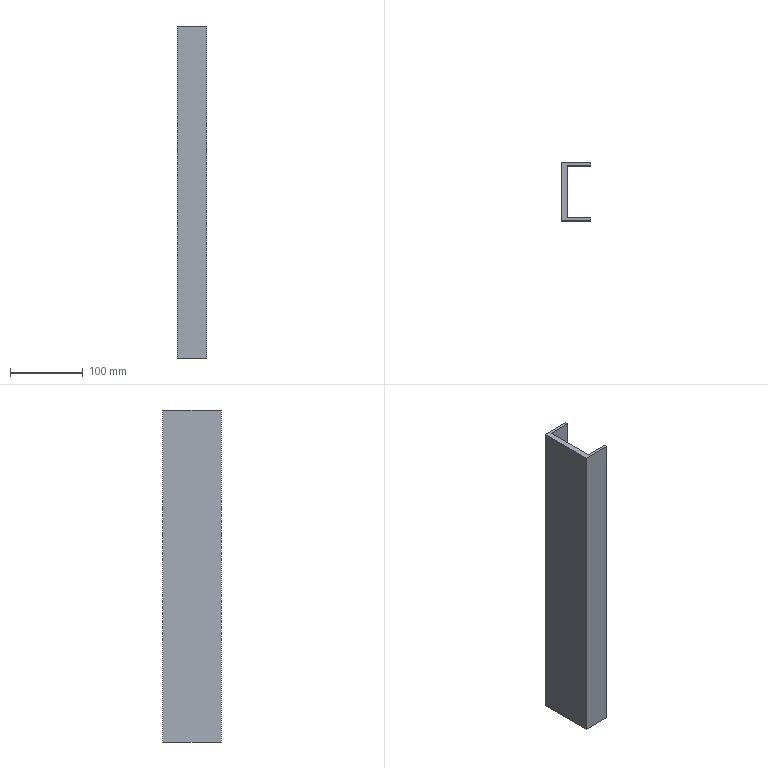Component | SolidWorks | BaseAssembly-1_ChannelSteelAssembly-1_8#ChannelSteel5-1 | 1 solid | 10 faces | box 40 x 80 x 455 mm | volume 407680 mm3 | plane 10
build123d program:
from build123d import *

# Parameters (mm, degrees)
EXTRUDE1_DEPTH = 455


with BuildPart() as part:
    # Sketch1 → Extrude1 (new body)
    with BuildSketch(Plane.XY):
        Polygon((0, 0), (-40, 0), (-40, 80), (0, 80), (0, 76), (-32, 76), (-32, 4), (0, 4), align=None)
    extrude(amount=EXTRUDE1_DEPTH)


solid = part.part

# Placed as in the assembly
solid = solid.moved(Location((-127.218, -82.9, -327.5), (0, 0, 0)))
STEP:
#1=COLOUR_RGB('',0.7922,0.8196,0.9333);
#2=FILL_AREA_STYLE_COLOUR('',#1);
#3=FILL_AREA_STYLE('',(#2));
#4=SURFACE_STYLE_FILL_AREA(#3);
#5=SURFACE_SIDE_STYLE('',(#4));
#6=SURFACE_STYLE_USAGE(.BOTH.,#5);
#7=PRESENTATION_STYLE_ASSIGNMENT((#6));
#8=CARTESIAN_POINT('',(-5.009,-0.1142,5.02));
#9=VERTEX_POINT('',#8);
#10=CARTESIAN_POINT('',(-5.009,-0.2717,5.02));
#11=VERTEX_POINT('',#10);
#12=CARTESIAN_POINT('',(-5.009,-0.2717,5.02));
#13=DIRECTION('',(0.,-1.,0.));
#14=VECTOR('',#13,39.37);
#15=LINE('',#12,#14);
#16=EDGE_CURVE('',#9,#11,#15,.T.);
#17=ORIENTED_EDGE('',*,*,#16,.T.);
#18=CARTESIAN_POINT('',(-5.009,-0.2717,-12.894));
#19=VERTEX_POINT('',#18);
#20=CARTESIAN_POINT('',(-5.009,-0.2717,-12.894));
#21=DIRECTION('',(-0.,0.,1.));
#22=VECTOR('',#21,39.37);
#23=LINE('',#20,#22);
#24=EDGE_CURVE('',#19,#11,#23,.T.);
#25=ORIENTED_EDGE('',*,*,#24,.F.);
#26=CARTESIAN_POINT('',(-5.009,-0.1142,-12.894));
#27=VERTEX_POINT('',#26);
#28=CARTESIAN_POINT('',(-5.009,-0.2717,-12.894));
#29=DIRECTION('',(0.,-1.,0.));
#30=VECTOR('',#29,39.37);
#31=LINE('',#28,#30);
#32=EDGE_CURVE('',#27,#19,#31,.T.);
#33=ORIENTED_EDGE('',*,*,#32,.F.);
#34=CARTESIAN_POINT('',(-5.009,-0.1142,-12.894));
#35=DIRECTION('',(-0.,0.,1.));
#36=VECTOR('',#35,39.37);
#37=LINE('',#34,#36);
#38=EDGE_CURVE('',#27,#9,#37,.T.);
#39=ORIENTED_EDGE('',*,*,#38,.T.);
#40=EDGE_LOOP('',(#17,#25,#33,#39));
#41=FACE_OUTER_BOUND('',#40,.T.);
#42=CARTESIAN_POINT('',(-5.009,-0.2717,-12.894));
#43=DIRECTION('',(-1.,-0.,-0.));
#44=DIRECTION('',(-0.,1.,-0.));
#45=AXIS2_PLACEMENT_3D('',#42,#43,#44);
#46=PLANE('',#45);
#47=ADVANCED_FACE('',(#41),#46,.F.);
#48=CARTESIAN_POINT('',(-6.268,-0.2717,5.02));
#49=VERTEX_POINT('',#48);
#50=CARTESIAN_POINT('',(-6.268,-0.2717,5.02));
#51=DIRECTION('',(-1.,-0.,-0.));
#52=VECTOR('',#51,39.37);
#53=LINE('',#50,#52);
#54=EDGE_CURVE('',#11,#49,#53,.T.);
#55=ORIENTED_EDGE('',*,*,#54,.T.);
#56=CARTESIAN_POINT('',(-6.268,-0.2717,-12.894));
#57=VERTEX_POINT('',#56);
#58=CARTESIAN_POINT('',(-6.268,-0.2717,-12.894));
#59=DIRECTION('',(-0.,0.,1.));
#60=VECTOR('',#59,39.37);
#61=LINE('',#58,#60);
#62=EDGE_CURVE('',#57,#49,#61,.T.);
#63=ORIENTED_EDGE('',*,*,#62,.F.);
#64=CARTESIAN_POINT('',(-6.268,-0.2717,-12.894));
#65=DIRECTION('',(-1.,-0.,-0.));
#66=VECTOR('',#65,39.37);
#67=LINE('',#64,#66);
#68=EDGE_CURVE('',#19,#57,#67,.T.);
#69=ORIENTED_EDGE('',*,*,#68,.F.);
#70=ORIENTED_EDGE('',*,*,#24,.T.);
#71=EDGE_LOOP('',(#55,#63,#69,#70));
#72=FACE_OUTER_BOUND('',#71,.T.);
#73=CARTESIAN_POINT('',(-6.268,-0.2717,-12.894));
#74=DIRECTION('',(-0.,1.,-0.));
#75=DIRECTION('',(-0.,0.,1.));
#76=AXIS2_PLACEMENT_3D('',#73,#74,#75);
#77=PLANE('',#76);
#78=ADVANCED_FACE('',(#72),#77,.F.);
#79=CARTESIAN_POINT('',(-6.268,-3.106,5.02));
#80=VERTEX_POINT('',#79);
#81=CARTESIAN_POINT('',(-6.268,-3.106,5.02));
#82=DIRECTION('',(0.,-1.,0.));
#83=VECTOR('',#82,39.37);
#84=LINE('',#81,#83);
#85=EDGE_CURVE('',#49,#80,#84,.T.);
#86=ORIENTED_EDGE('',*,*,#85,.T.);
#87=CARTESIAN_POINT('',(-6.268,-3.106,-12.894));
#88=VERTEX_POINT('',#87);
#89=CARTESIAN_POINT('',(-6.268,-3.106,-12.894));
#90=DIRECTION('',(-0.,0.,1.));
#91=VECTOR('',#90,39.37);
#92=LINE('',#89,#91);
#93=EDGE_CURVE('',#88,#80,#92,.T.);
#94=ORIENTED_EDGE('',*,*,#93,.F.);
#95=CARTESIAN_POINT('',(-6.268,-3.106,-12.894));
#96=DIRECTION('',(0.,-1.,0.));
#97=VECTOR('',#96,39.37);
#98=LINE('',#95,#97);
#99=EDGE_CURVE('',#57,#88,#98,.T.);
#100=ORIENTED_EDGE('',*,*,#99,.F.);
#101=ORIENTED_EDGE('',*,*,#62,.T.);
#102=EDGE_LOOP('',(#86,#94,#100,#101));
#103=FACE_OUTER_BOUND('',#102,.T.);
#104=CARTESIAN_POINT('',(-6.268,-3.106,-12.894));
#105=DIRECTION('',(-1.,-0.,-0.));
#106=DIRECTION('',(-0.,1.,-0.));
#107=AXIS2_PLACEMENT_3D('',#104,#105,#106);
#108=PLANE('',#107);
#109=ADVANCED_FACE('',(#103),#108,.F.);
#110=CARTESIAN_POINT('',(-5.009,-3.106,5.02));
#111=VERTEX_POINT('',#110);
#112=CARTESIAN_POINT('',(-5.009,-3.106,5.02));
#113=DIRECTION('',(1.,0.,0.));
#114=VECTOR('',#113,39.37);
#115=LINE('',#112,#114);
#116=EDGE_CURVE('',#80,#111,#115,.T.);
#117=ORIENTED_EDGE('',*,*,#116,.T.);
#118=CARTESIAN_POINT('',(-5.009,-3.106,-12.894));
#119=VERTEX_POINT('',#118);
#120=CARTESIAN_POINT('',(-5.009,-3.106,-12.894));
#121=DIRECTION('',(-0.,0.,1.));
#122=VECTOR('',#121,39.37);
#123=LINE('',#120,#122);
#124=EDGE_CURVE('',#119,#111,#123,.T.);
#125=ORIENTED_EDGE('',*,*,#124,.F.);
#126=CARTESIAN_POINT('',(-5.009,-3.106,-12.894));
#127=DIRECTION('',(1.,0.,0.));
#128=VECTOR('',#127,39.37);
#129=LINE('',#126,#128);
#130=EDGE_CURVE('',#88,#119,#129,.T.);
#131=ORIENTED_EDGE('',*,*,#130,.F.);
#132=ORIENTED_EDGE('',*,*,#93,.T.);
#133=EDGE_LOOP('',(#117,#125,#131,#132));
#134=FACE_OUTER_BOUND('',#133,.T.);
#135=CARTESIAN_POINT('',(-5.009,-3.106,-12.894));
#136=DIRECTION('',(0.,-1.,0.));
#137=DIRECTION('',(0.,-0.,-1.));
#138=AXIS2_PLACEMENT_3D('',#135,#136,#137);
#139=PLANE('',#138);
#140=ADVANCED_FACE('',(#134),#139,.F.);
#141=CARTESIAN_POINT('',(-5.009,-3.264,5.02));
#142=VERTEX_POINT('',#141);
#143=CARTESIAN_POINT('',(-5.009,-3.264,5.02));
#144=DIRECTION('',(0.,-1.,0.));
#145=VECTOR('',#144,39.37);
#146=LINE('',#143,#145);
#147=EDGE_CURVE('',#111,#142,#146,.T.);
#148=ORIENTED_EDGE('',*,*,#147,.T.);
#149=CARTESIAN_POINT('',(-5.009,-3.264,-12.894));
#150=VERTEX_POINT('',#149);
#151=CARTESIAN_POINT('',(-5.009,-3.264,-12.894));
#152=DIRECTION('',(-0.,0.,1.));
#153=VECTOR('',#152,39.37);
#154=LINE('',#151,#153);
#155=EDGE_CURVE('',#150,#142,#154,.T.);
#156=ORIENTED_EDGE('',*,*,#155,.F.);
#157=CARTESIAN_POINT('',(-5.009,-3.264,-12.894));
#158=DIRECTION('',(0.,-1.,0.));
#159=VECTOR('',#158,39.37);
#160=LINE('',#157,#159);
#161=EDGE_CURVE('',#119,#150,#160,.T.);
#162=ORIENTED_EDGE('',*,*,#161,.F.);
#163=ORIENTED_EDGE('',*,*,#124,.T.);
#164=EDGE_LOOP('',(#148,#156,#162,#163));
#165=FACE_OUTER_BOUND('',#164,.T.);
#166=CARTESIAN_POINT('',(-5.009,-3.264,-12.894));
#167=DIRECTION('',(-1.,-0.,-0.));
#168=DIRECTION('',(0.,-0.,-1.));
#169=AXIS2_PLACEMENT_3D('',#166,#167,#168);
#170=PLANE('',#169);
#171=ADVANCED_FACE('',(#165),#170,.F.);
#172=CARTESIAN_POINT('',(-6.583,-3.264,5.02));
#173=VERTEX_POINT('',#172);
#174=CARTESIAN_POINT('',(-6.583,-3.264,5.02));
#175=DIRECTION('',(-1.,-0.,-0.));
#176=VECTOR('',#175,39.37);
#177=LINE('',#174,#176);
#178=EDGE_CURVE('',#142,#173,#177,.T.);
#179=ORIENTED_EDGE('',*,*,#178,.T.);
#180=CARTESIAN_POINT('',(-6.583,-3.264,-12.894));
#181=VERTEX_POINT('',#180);
#182=CARTESIAN_POINT('',(-6.583,-3.264,-12.894));
#183=DIRECTION('',(-0.,0.,1.));
#184=VECTOR('',#183,39.37);
#185=LINE('',#182,#184);
#186=EDGE_CURVE('',#181,#173,#185,.T.);
#187=ORIENTED_EDGE('',*,*,#186,.F.);
#188=CARTESIAN_POINT('',(-6.583,-3.264,-12.894));
#189=DIRECTION('',(-1.,-0.,-0.));
#190=VECTOR('',#189,39.37);
#191=LINE('',#188,#190);
#192=EDGE_CURVE('',#150,#181,#191,.T.);
#193=ORIENTED_EDGE('',*,*,#192,.F.);
#194=ORIENTED_EDGE('',*,*,#155,.T.);
#195=EDGE_LOOP('',(#179,#187,#193,#194));
#196=FACE_OUTER_BOUND('',#195,.T.);
#197=CARTESIAN_POINT('',(-6.583,-3.264,-12.894));
#198=DIRECTION('',(-0.,1.,-0.));
#199=DIRECTION('',(-0.,0.,1.));
#200=AXIS2_PLACEMENT_3D('',#197,#198,#199);
#201=PLANE('',#200);
#202=ADVANCED_FACE('',(#196),#201,.F.);
#203=CARTESIAN_POINT('',(-6.583,-0.1142,5.02));
#204=VERTEX_POINT('',#203);
#205=CARTESIAN_POINT('',(-6.583,-0.1142,5.02));
#206=DIRECTION('',(-0.,1.,-0.));
#207=VECTOR('',#206,39.37);
#208=LINE('',#205,#207);
#209=EDGE_CURVE('',#173,#204,#208,.T.);
#210=ORIENTED_EDGE('',*,*,#209,.T.);
#211=CARTESIAN_POINT('',(-6.583,-0.1142,-12.894));
#212=VERTEX_POINT('',#211);
#213=CARTESIAN_POINT('',(-6.583,-0.1142,-12.894));
#214=DIRECTION('',(-0.,0.,1.));
#215=VECTOR('',#214,39.37);
#216=LINE('',#213,#215);
#217=EDGE_CURVE('',#212,#204,#216,.T.);
#218=ORIENTED_EDGE('',*,*,#217,.F.);
#219=CARTESIAN_POINT('',(-6.583,-0.1142,-12.894));
#220=DIRECTION('',(-0.,1.,-0.));
#221=VECTOR('',#220,39.37);
#222=LINE('',#219,#221);
#223=EDGE_CURVE('',#181,#212,#222,.T.);
#224=ORIENTED_EDGE('',*,*,#223,.F.);
#225=ORIENTED_EDGE('',*,*,#186,.T.);
#226=EDGE_LOOP('',(#210,#218,#224,#225));
#227=FACE_OUTER_BOUND('',#226,.T.);
#228=CARTESIAN_POINT('',(-6.583,-0.1142,-12.894));
#229=DIRECTION('',(1.,0.,0.));
#230=DIRECTION('',(-0.,0.,1.));
#231=AXIS2_PLACEMENT_3D('',#228,#229,#230);
#232=PLANE('',#231);
#233=ADVANCED_FACE('',(#227),#232,.F.);
#234=CARTESIAN_POINT('',(-5.009,-0.1142,5.02));
#235=DIRECTION('',(1.,0.,0.));
#236=VECTOR('',#235,39.37);
#237=LINE('',#234,#236);
#238=EDGE_CURVE('',#204,#9,#237,.T.);
#239=ORIENTED_EDGE('',*,*,#238,.T.);
#240=ORIENTED_EDGE('',*,*,#38,.F.);
#241=CARTESIAN_POINT('',(-5.009,-0.1142,-12.894));
#242=DIRECTION('',(1.,0.,0.));
#243=VECTOR('',#242,39.37);
#244=LINE('',#241,#243);
#245=EDGE_CURVE('',#212,#27,#244,.T.);
#246=ORIENTED_EDGE('',*,*,#245,.F.);
#247=ORIENTED_EDGE('',*,*,#217,.T.);
#248=EDGE_LOOP('',(#239,#240,#246,#247));
#249=FACE_OUTER_BOUND('',#248,.T.);
#250=CARTESIAN_POINT('',(-5.009,-0.1142,-12.894));
#251=DIRECTION('',(0.,-1.,0.));
#252=DIRECTION('',(-1.,-0.,-0.));
#253=AXIS2_PLACEMENT_3D('',#250,#251,#252);
#254=PLANE('',#253);
#255=ADVANCED_FACE('',(#249),#254,.F.);
#256=ORIENTED_EDGE('',*,*,#32,.T.);
#257=ORIENTED_EDGE('',*,*,#68,.T.);
#258=ORIENTED_EDGE('',*,*,#99,.T.);
#259=ORIENTED_EDGE('',*,*,#130,.T.);
#260=ORIENTED_EDGE('',*,*,#161,.T.);
#261=ORIENTED_EDGE('',*,*,#192,.T.);
#262=ORIENTED_EDGE('',*,*,#223,.T.);
#263=ORIENTED_EDGE('',*,*,#245,.T.);
#264=EDGE_LOOP('',(#256,#257,#258,#259,#260,#261,#262,#263));
#265=FACE_OUTER_BOUND('',#264,.T.);
#266=CARTESIAN_POINT('',(-5.009,-3.264,-12.894));
#267=DIRECTION('',(0.,-0.,-1.));
#268=DIRECTION('',(1.,0.,0.));
#269=AXIS2_PLACEMENT_3D('',#266,#267,#268);
#270=PLANE('',#269);
#271=ADVANCED_FACE('',(#265),#270,.T.);
#272=ORIENTED_EDGE('',*,*,#16,.F.);
#273=ORIENTED_EDGE('',*,*,#238,.F.);
#274=ORIENTED_EDGE('',*,*,#209,.F.);
#275=ORIENTED_EDGE('',*,*,#178,.F.);
#276=ORIENTED_EDGE('',*,*,#147,.F.);
#277=ORIENTED_EDGE('',*,*,#116,.F.);
#278=ORIENTED_EDGE('',*,*,#85,.F.);
#279=ORIENTED_EDGE('',*,*,#54,.F.);
#280=EDGE_LOOP('',(#272,#273,#274,#275,#276,#277,#278,#279));
#281=FACE_OUTER_BOUND('',#280,.T.);
#282=CARTESIAN_POINT('',(-5.009,-3.264,5.02));
#283=DIRECTION('',(0.,-0.,-1.));
#284=DIRECTION('',(1.,0.,0.));
#285=AXIS2_PLACEMENT_3D('',#282,#283,#284);
#286=PLANE('',#285);
#287=ADVANCED_FACE('',(#281),#286,.F.);
#288=CLOSED_SHELL('',(#47,#78,#109,#140,#171,#202,#233,#255,#271,#287));
#289=MANIFOLD_SOLID_BREP('',#288);
#290=STYLED_ITEM('',(#7),#289);
#291=PRESENTATION_LAYER_ASSIGNMENT('','',(#290));
#292=(LENGTH_UNIT()NAMED_UNIT(*)SI_UNIT($,.METRE.));
#293=LENGTH_MEASURE_WITH_UNIT(LENGTH_MEASURE(0.0254),#292);
#294=DIMENSIONAL_EXPONENTS(1.,0.,0.,0.,0.,0.,0.);
#295=(CONVERSION_BASED_UNIT('',#293)LENGTH_UNIT()NAMED_UNIT(#294));
#296=UNCERTAINTY_MEASURE_WITH_UNIT(LENGTH_MEASURE(0.00001),#295,'','');
#297=(NAMED_UNIT(*)PLANE_ANGLE_UNIT()SI_UNIT($,.RADIAN.));
#298=(NAMED_UNIT(*)SI_UNIT($,.STERADIAN.)SOLID_ANGLE_UNIT());
#299=(GEOMETRIC_REPRESENTATION_CONTEXT(3)GLOBAL_UNCERTAINTY_ASSIGNED_CONTEXT((#296))GLOBAL_UNIT_ASSIGNED_CONTEXT((#295,#297,#298))REPRESENTATION_CONTEXT('',''));
#300=MECHANICAL_DESIGN_GEOMETRIC_PRESENTATION_REPRESENTATION('',(#290),#299);
#301=CARTESIAN_POINT('',(0.,0.,0.));
#302=DIRECTION('',(0.,0.,1.));
#303=DIRECTION('',(1.,0.,0.));
#304=AXIS2_PLACEMENT_3D('',#301,#302,#303);
#305=(LENGTH_UNIT()NAMED_UNIT(*)SI_UNIT($,.METRE.));
#306=LENGTH_MEASURE_WITH_UNIT(LENGTH_MEASURE(0.0254),#305);
#307=DIMENSIONAL_EXPONENTS(1.,0.,0.,0.,0.,0.,0.);
#308=(CONVERSION_BASED_UNIT('',#306)LENGTH_UNIT()NAMED_UNIT(#307));
#309=UNCERTAINTY_MEASURE_WITH_UNIT(LENGTH_MEASURE(0.00001),#308,'','');
#310=(NAMED_UNIT(*)PLANE_ANGLE_UNIT()SI_UNIT($,.RADIAN.));
#311=(NAMED_UNIT(*)SI_UNIT($,.STERADIAN.)SOLID_ANGLE_UNIT());
#312=(GEOMETRIC_REPRESENTATION_CONTEXT(3)GLOBAL_UNCERTAINTY_ASSIGNED_CONTEXT((#309))GLOBAL_UNIT_ASSIGNED_CONTEXT((#308,#310,#311))REPRESENTATION_CONTEXT('',''));
#313=ADVANCED_BREP_SHAPE_REPRESENTATION('',(#289,#304),#312);